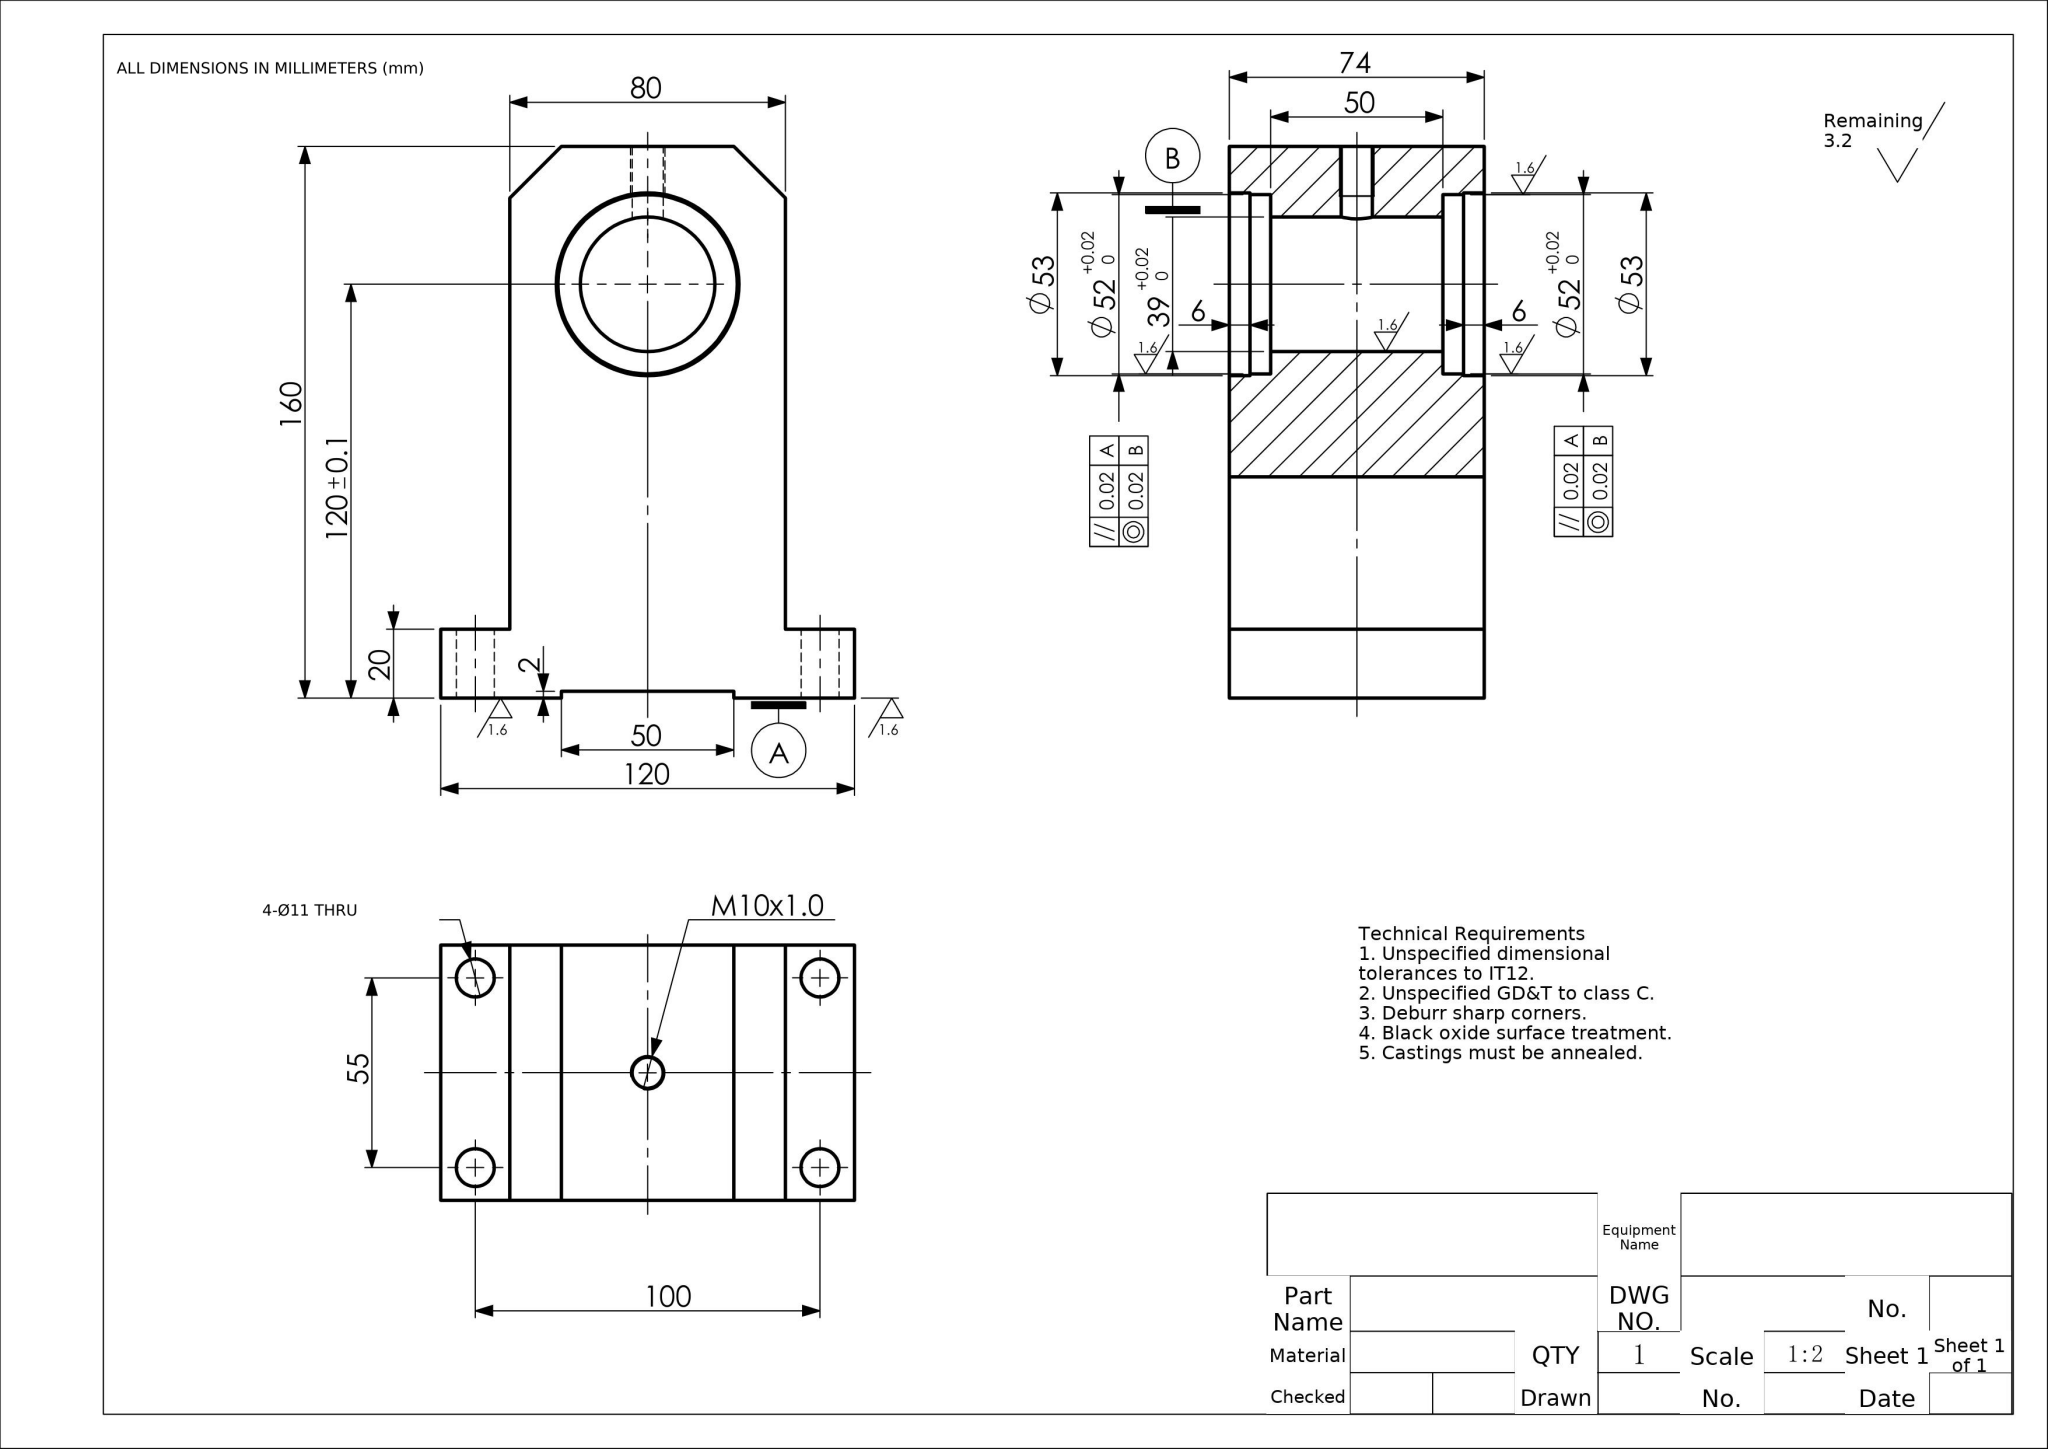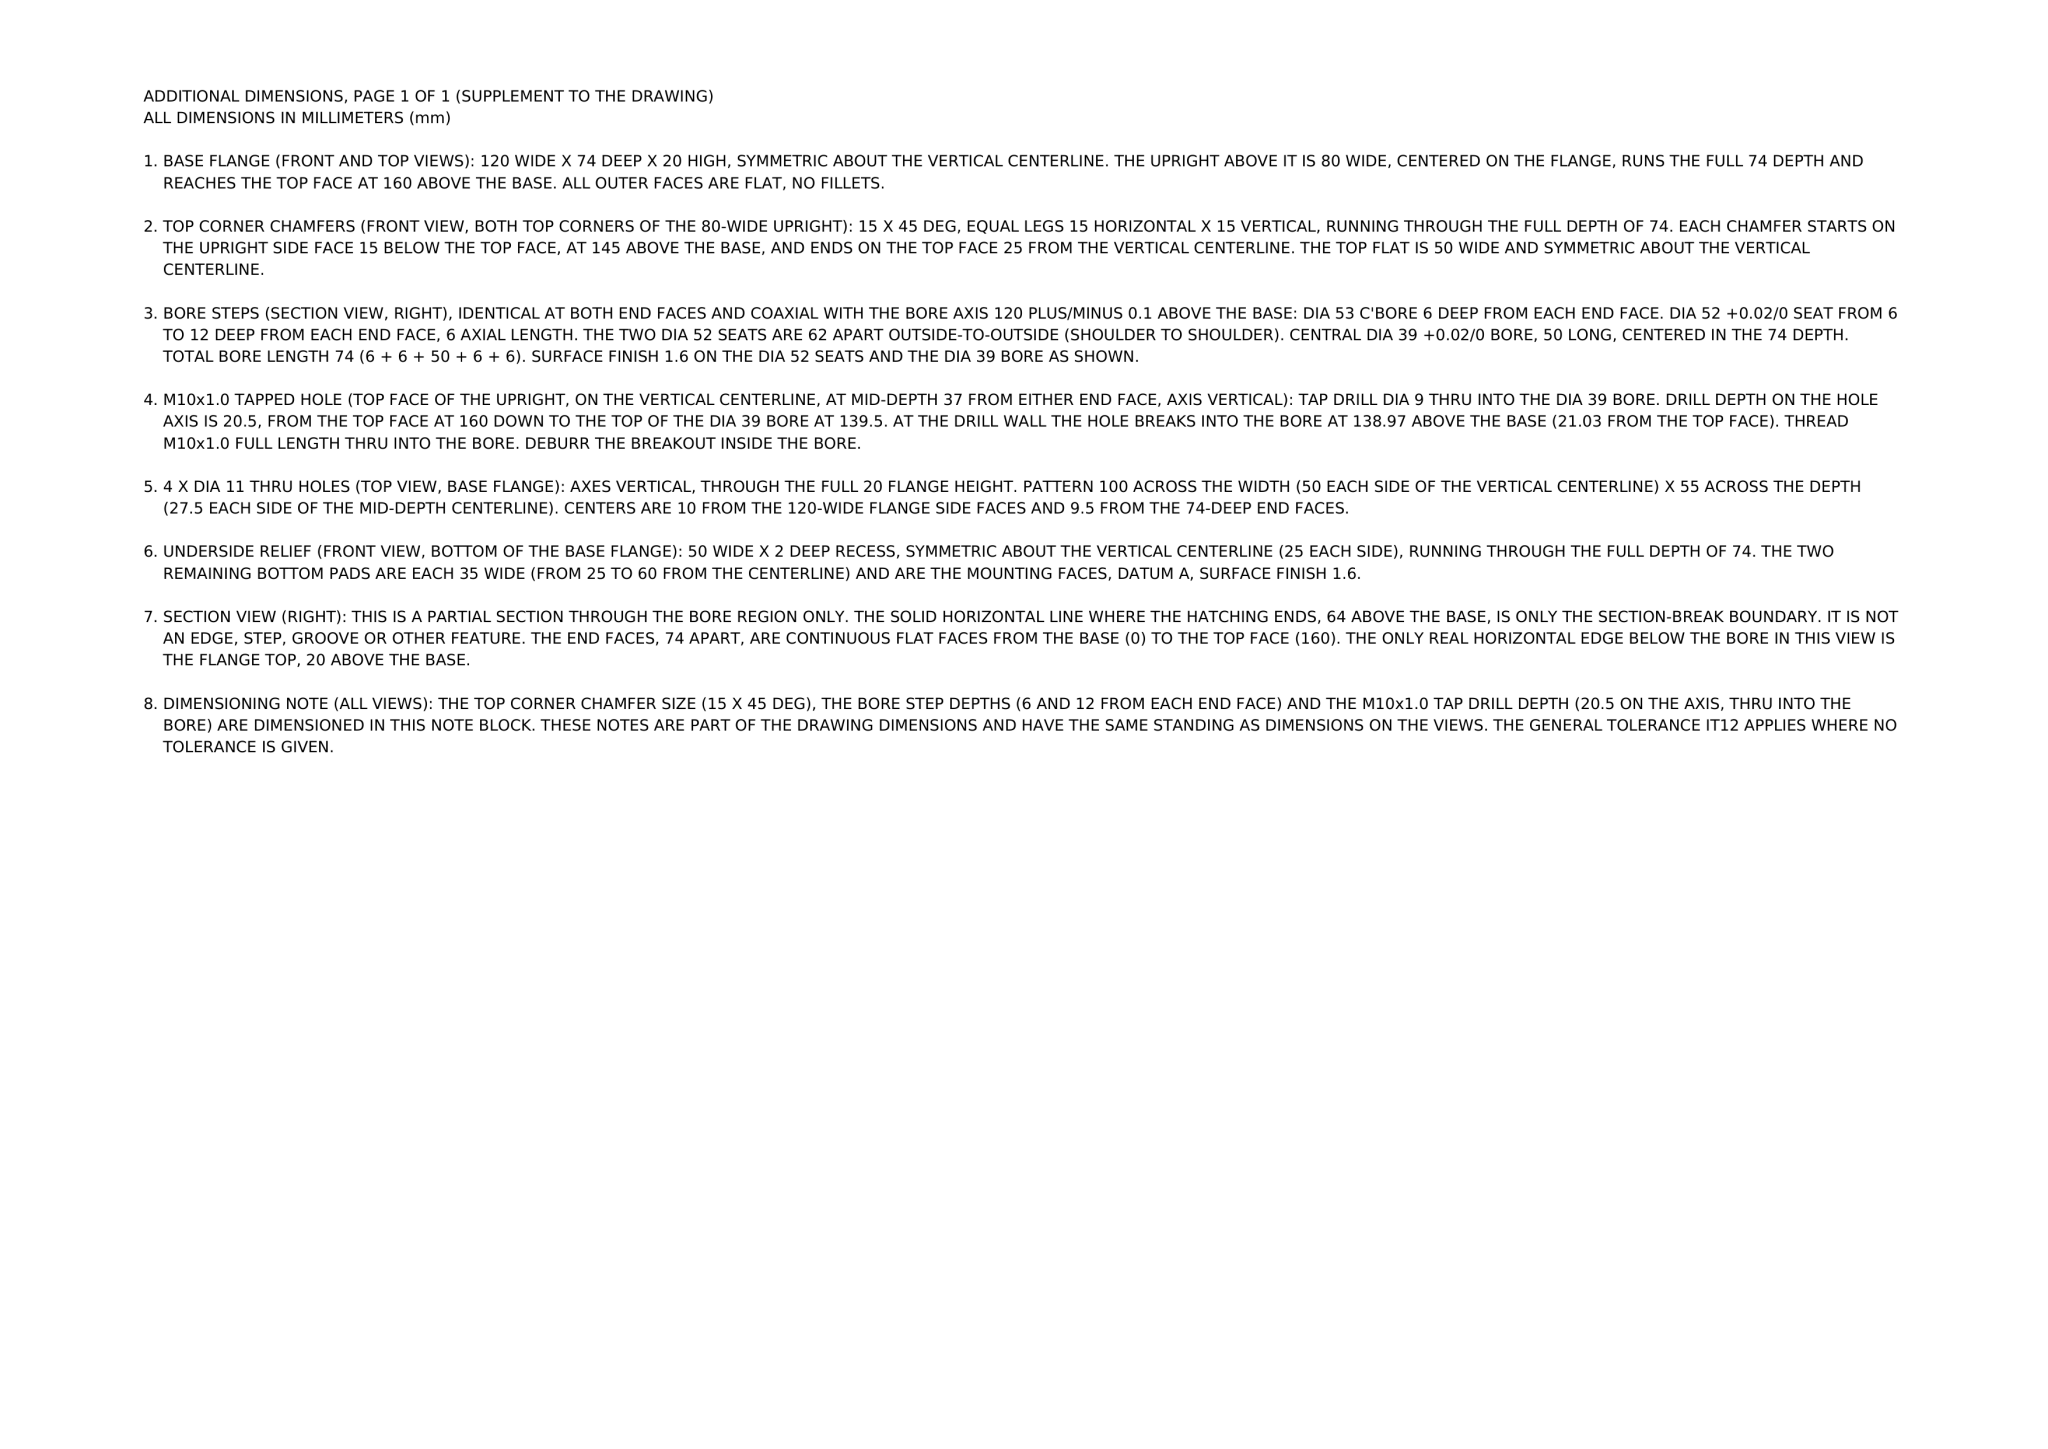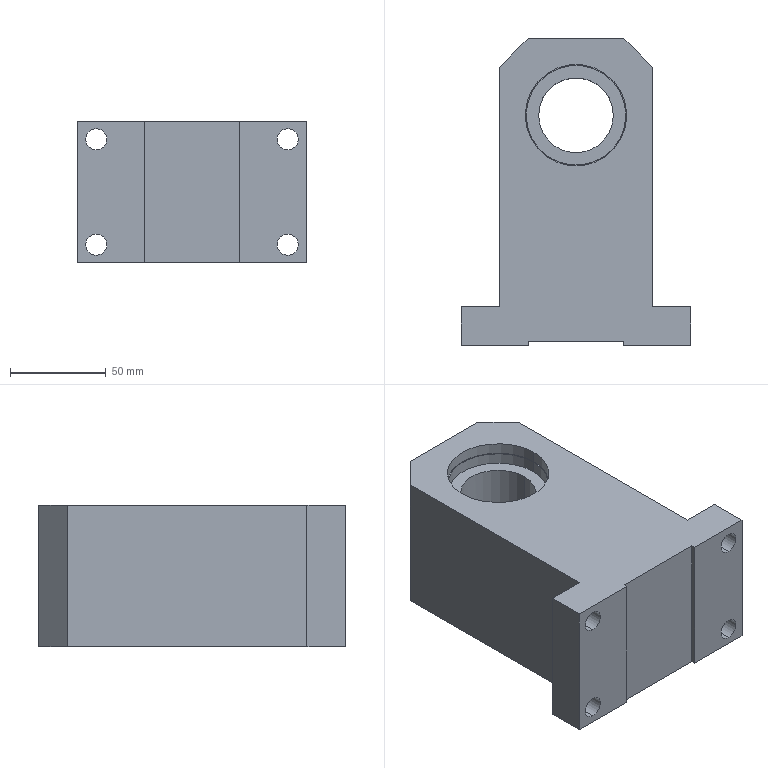Part | NX | mm | 1 solid | 40 faces | box 120 x 160 x 74 mm | volume 861747 mm3 | cylinder 20 | plane 20 | commonest cylinder face diameters 11 x8 53 x4 52 x4 9 x2 39 x2